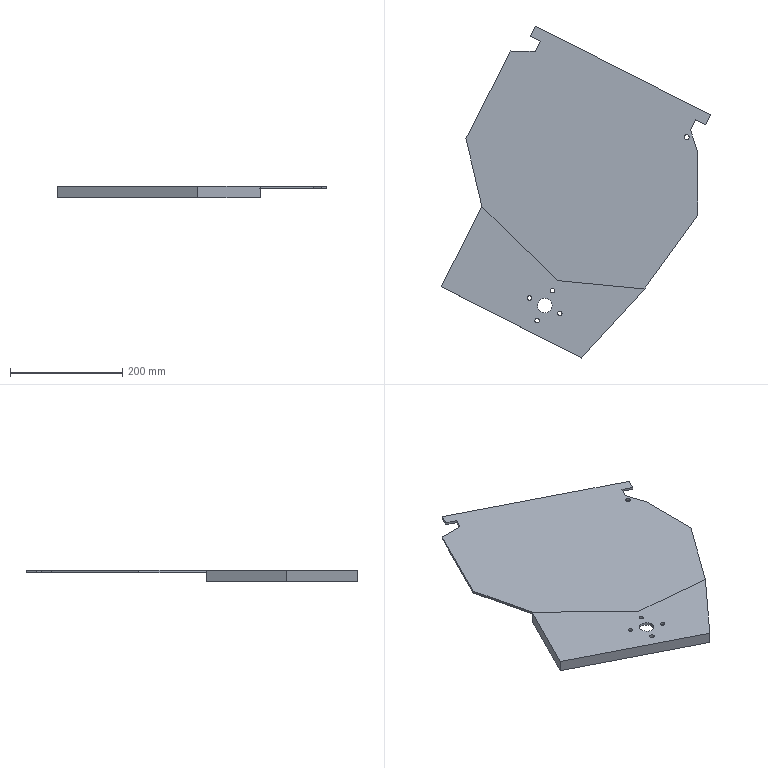Component | SolidWorks | SeedBoxAssemblyModified-1_SeedBoxLidModificationOtherSide-1 | 2 solids | 42 faces | box 479.48 x 590.78 x 20 mm | volume 805703 mm3 | plane 30 | cylinder 12 | commonest cylinder face diameters 8 x8 26 x2 9 x2
build123d program:
from build123d import *

# Parameters (mm, degrees)
BOSS_EXTRUDE2_DEPTH = 4
BOSS_EXTRUDE3_DEPTH = 20
SHELL1_T            = -5
SKETCH3_R           = 4.5
CUT_EXTRUDE1_DEPTH  = 578.016
SKETCH4_R           = 13
CUT_EXTRUDE2_DEPTH  = 578.016
SKETCH6_R           = 4
CUT_EXTRUDE3_DEPTH  = 578.016


with BuildPart() as part:
    # Sketch1 → Boss-Extrude2 (new body)
    with BuildSketch(Plane.XY):
        Polygon((-49.308, 39.622), (300.692, 39.622), (300.692, 19.622), (280.692, 19.622), (280.692, -0.3785), (310.55, -30.065), (360.55, -130.065), (335.55, -290.057), (190.657, -346.682), (11.335, -290.057), (-68.665, -195.057), (-68.665, -20.057), (-29.308, -0.3785), (-29.308, 19.622), (-49.308, 19.622), align=None)
    extrude(amount=-BOSS_EXTRUDE2_DEPTH)

    # Sketch3 → Cut-Extrude1 (cut, through all)
    with BuildSketch(Plane.XY):
        with Locations((280.55, -15.065)):
            Circle(SKETCH3_R)
    extrude(amount=-CUT_EXTRUDE1_DEPTH, mode=Mode.SUBTRACT)


with BuildPart() as body_2:
    # Sketch2 → Boss-Extrude3 (new body)
    with BuildSketch(Plane.XY):
        Polygon((11.335, -290.057), (11.335, -450.057), (291.335, -450.057), (335.55, -290.057), (190.657, -346.682), align=None)
    extrude(amount=-BOSS_EXTRUDE3_DEPTH)

    # Shell1
    shell1_openings = [body_2.faces().sort_by_distance(p)[0] for p in [
        (158.785, -381.977, -20),
    ]]
    offset(amount=SHELL1_T, openings=shell1_openings, kind=Kind.INTERSECTION)

    # Sketch4 → Cut-Extrude2 (cut, through all)
    with BuildSketch(Plane.XY):
        with Locations((190.657, -396.682)):
            Circle(SKETCH4_R)
    extrude(amount=-CUT_EXTRUDE2_DEPTH, mode=Mode.SUBTRACT)

    # Sketch6 → Cut-Extrude3 (cut, through all)
    with BuildSketch(Plane.XY):
        with Locations((190.657, -366.682)):
            Circle(SKETCH6_R)
        with Locations((160.657, -396.682)):
            Circle(SKETCH6_R)
        with Locations((190.657, -426.682)):
            Circle(SKETCH6_R)
        with Locations((220.657, -396.682)):
            Circle(SKETCH6_R)
    extrude(amount=-CUT_EXTRUDE3_DEPTH, mode=Mode.SUBTRACT)


solid = Compound([part.part, body_2.part])

# Placed as in the assembly
solid = solid.moved(Location((240.361, -400.339, 2462.971), (0, 0, -26.879)))